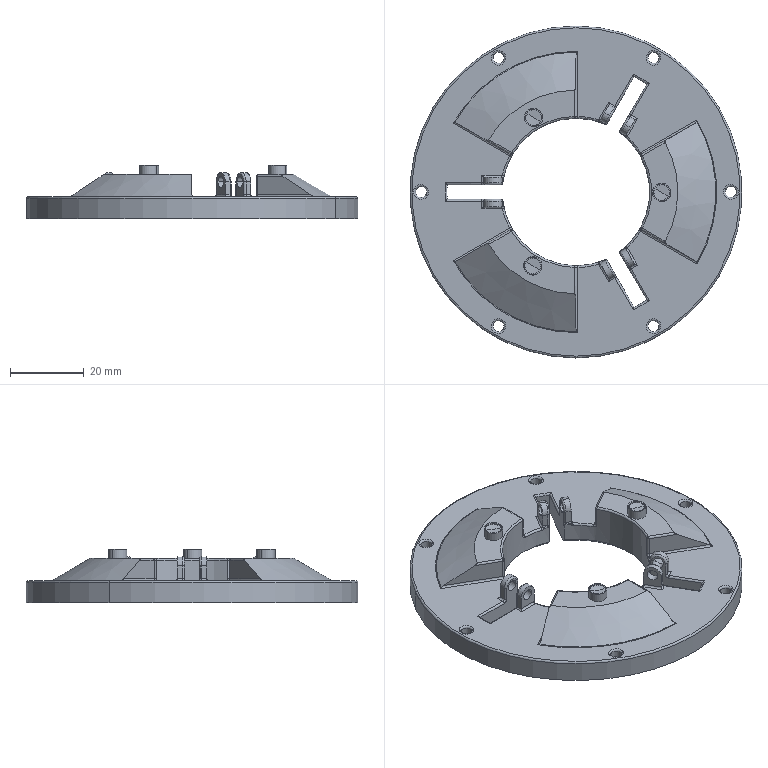Component | SolidWorks | JawCover-1 | 1 solid | 243 faces | volume 36068 mm3 | cylinder 116 | torus 48 | plane 41 | spline 18 | sphere 13 | cone 7 | commonest cylinder face diameters 1 x57 3 x24 5 x14 4.225 x6 4.6 x6 40 x4 70 x3 90 x2